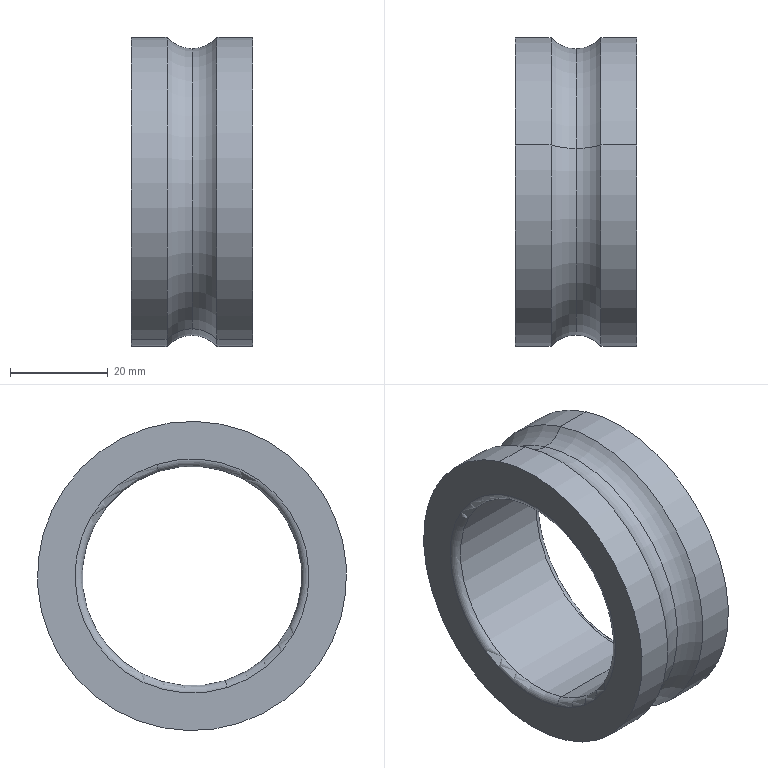Component | SolidWorks | UpperHousingAssembly-1_WormAxisAssembly-1_DeepGrooveBallBearing6309-1_BearingInnerRing-1 | 1 solid | 16 faces | box 25 x 63.4 x 63.4 mm | volume 35870 mm3 | torus 8 | cylinder 6 | plane 2 | commonest cylinder face diameters 63.4 x4 45 x2
build123d program:
from build123d import *

# Parameters (mm, degrees)
FILLET1_R = 1.5


with BuildPart() as part:
    # Sketch1 → Revolve1 (revolve)
    with BuildSketch(Plane.XY, mode=Mode.PRIVATE) as revolve1_sk:
        with BuildLine():
            Line((5.121, 31.7), (12.5, 31.7))
            Line((12.5, 31.7), (12.5, 22.5))
            Line((12.5, 22.5), (-12.5, 22.5))
            Line((-12.5, 22.5), (-12.5, 31.7))
            Line((-12.5, 31.7), (-5.121, 31.7))
            ThreePointArc((-5.121, 31.7), (0, 29.4), (5.121, 31.7))
        make_face()
    revolve(revolve1_sk.sketch.rotate(Axis((-18.919, 0, 0), (1, 0, 0)), 90), axis=Axis((-18.919, 0, 0), (1, 0, 0)))

    # Fillet1
    fillet1_edges = [part.edges().sort_by_distance(p)[0] for p in [
        (12.5, 0, -22.5),
        (-12.5, 0, -22.5),
    ]]
    fillet(fillet1_edges, radius=FILLET1_R)


solid = part.part

# Placed as in the assembly
solid = solid.moved(Location((1019.077, 1408.591, 1694.217), (0, 0, 0)))
STEP:
#1=COLOUR_RGB('',0.7922,0.8196,0.9333);
#2=FILL_AREA_STYLE_COLOUR('',#1);
#3=FILL_AREA_STYLE('',(#2));
#4=SURFACE_STYLE_FILL_AREA(#3);
#5=SURFACE_SIDE_STYLE('',(#4));
#6=SURFACE_STYLE_USAGE(.BOTH.,#5);
#7=PRESENTATION_STYLE_ASSIGNMENT((#6));
#8=CARTESIAN_POINT('',(39.92,55.834,67.891));
#9=VERTEX_POINT('',#8);
#10=CARTESIAN_POINT('',(40.121,55.806,67.805));
#11=VERTEX_POINT('',#10);
#12=CARTESIAN_POINT('',(40.121,55.888,68.062));
#13=DIRECTION('',(0.,-0.9532,0.3024));
#14=DIRECTION('',(0.,-0.3024,-0.9532));
#15=AXIS2_PLACEMENT_3D('',#12,#13,#14);
#16=CIRCLE('',#15,0.2697);
#17=EDGE_CURVE('',#9,#11,#16,.T.);
#18=ORIENTED_EDGE('',*,*,#17,.T.);
#19=CARTESIAN_POINT('',(40.121,55.106,65.598));
#20=VERTEX_POINT('',#19);
#21=CARTESIAN_POINT('',(40.121,55.456,66.701));
#22=DIRECTION('',(-1.,0.,0.));
#23=DIRECTION('',(0.,0.,1.));
#24=AXIS2_PLACEMENT_3D('',#21,#22,#23);
#25=CIRCLE('',#24,1.157);
#26=EDGE_CURVE('',#11,#20,#25,.T.);
#27=ORIENTED_EDGE('',*,*,#26,.T.);
#28=CARTESIAN_POINT('',(39.92,55.079,65.512));
#29=VERTEX_POINT('',#28);
#30=CARTESIAN_POINT('',(40.121,55.025,65.341));
#31=DIRECTION('',(0.,0.9532,-0.3024));
#32=DIRECTION('',(0.,0.3024,0.9532));
#33=AXIS2_PLACEMENT_3D('',#30,#31,#32);
#34=CIRCLE('',#33,0.2697);
#35=EDGE_CURVE('',#29,#20,#34,.T.);
#36=ORIENTED_EDGE('',*,*,#35,.F.);
#37=CARTESIAN_POINT('',(39.92,55.456,66.701));
#38=DIRECTION('',(-1.,0.,0.));
#39=DIRECTION('',(0.,0.3024,0.9532));
#40=AXIS2_PLACEMENT_3D('',#37,#38,#39);
#41=CIRCLE('',#40,1.248);
#42=EDGE_CURVE('',#9,#29,#41,.T.);
#43=ORIENTED_EDGE('',*,*,#42,.F.);
#44=EDGE_LOOP('',(#18,#27,#36,#43));
#45=FACE_OUTER_BOUND('',#44,.T.);
#46=CARTESIAN_POINT('',(40.121,55.456,66.701));
#47=DIRECTION('',(-1.,0.,0.));
#48=DIRECTION('',(0.,0.3024,0.9532));
#49=AXIS2_PLACEMENT_3D('',#46,#47,#48);
#50=TOROIDAL_SURFACE('',#49,1.427,0.2697);
#51=ADVANCED_FACE('',(#45),#50,.F.);
#52=ORIENTED_EDGE('',*,*,#35,.T.);
#53=CARTESIAN_POINT('',(40.121,55.456,66.701));
#54=DIRECTION('',(-1.,0.,0.));
#55=DIRECTION('',(0.,0.,1.));
#56=AXIS2_PLACEMENT_3D('',#53,#54,#55);
#57=CIRCLE('',#56,1.157);
#58=EDGE_CURVE('',#20,#11,#57,.T.);
#59=ORIENTED_EDGE('',*,*,#58,.T.);
#60=ORIENTED_EDGE('',*,*,#17,.F.);
#61=CARTESIAN_POINT('',(39.92,55.456,66.701));
#62=DIRECTION('',(-1.,0.,0.));
#63=DIRECTION('',(0.,0.3024,0.9532));
#64=AXIS2_PLACEMENT_3D('',#61,#62,#63);
#65=CIRCLE('',#64,1.248);
#66=EDGE_CURVE('',#29,#9,#65,.T.);
#67=ORIENTED_EDGE('',*,*,#66,.F.);
#68=EDGE_LOOP('',(#52,#59,#60,#67));
#69=FACE_OUTER_BOUND('',#68,.T.);
#70=CARTESIAN_POINT('',(40.121,55.456,66.701));
#71=DIRECTION('',(-1.,0.,0.));
#72=DIRECTION('',(0.,0.3024,0.9532));
#73=AXIS2_PLACEMENT_3D('',#70,#71,#72);
#74=TOROIDAL_SURFACE('',#73,1.427,0.2697);
#75=ADVANCED_FACE('',(#69),#74,.F.);
#76=CARTESIAN_POINT('',(40.554,55.188,65.857));
#77=VERTEX_POINT('',#76);
#78=CARTESIAN_POINT('',(40.554,55.724,67.546));
#79=VERTEX_POINT('',#78);
#80=CARTESIAN_POINT('',(40.554,55.456,66.701));
#81=DIRECTION('',(1.,0.,0.));
#82=DIRECTION('',(0.,0.3024,0.9532));
#83=AXIS2_PLACEMENT_3D('',#80,#81,#82);
#84=CIRCLE('',#83,0.8858);
#85=EDGE_CURVE('',#77,#79,#84,.T.);
#86=ORIENTED_EDGE('',*,*,#85,.F.);
#87=CARTESIAN_POINT('',(40.613,55.171,65.801));
#88=VERTEX_POINT('',#87);
#89=CARTESIAN_POINT('',(40.554,55.171,65.801));
#90=DIRECTION('',(0.,0.9532,-0.3024));
#91=DIRECTION('',(0.,0.3024,0.9532));
#92=AXIS2_PLACEMENT_3D('',#89,#90,#91);
#93=CIRCLE('',#92,0.05906);
#94=EDGE_CURVE('',#77,#88,#93,.T.);
#95=ORIENTED_EDGE('',*,*,#94,.T.);
#96=CARTESIAN_POINT('',(40.613,55.742,67.602));
#97=VERTEX_POINT('',#96);
#98=CARTESIAN_POINT('',(40.613,55.456,66.701));
#99=DIRECTION('',(-1.,0.,0.));
#100=DIRECTION('',(0.,0.3024,0.9532));
#101=AXIS2_PLACEMENT_3D('',#98,#99,#100);
#102=CIRCLE('',#101,0.9449);
#103=EDGE_CURVE('',#97,#88,#102,.T.);
#104=ORIENTED_EDGE('',*,*,#103,.F.);
#105=CARTESIAN_POINT('',(40.554,55.742,67.602));
#106=DIRECTION('',(0.,-0.9532,0.3024));
#107=DIRECTION('',(0.,-0.3024,-0.9532));
#108=AXIS2_PLACEMENT_3D('',#105,#106,#107);
#109=CIRCLE('',#108,0.05906);
#110=EDGE_CURVE('',#79,#97,#109,.T.);
#111=ORIENTED_EDGE('',*,*,#110,.F.);
#112=EDGE_LOOP('',(#86,#95,#104,#111));
#113=FACE_OUTER_BOUND('',#112,.T.);
#114=CARTESIAN_POINT('',(40.554,55.456,66.701));
#115=DIRECTION('',(-1.,0.,0.));
#116=DIRECTION('',(0.,0.3024,0.9532));
#117=AXIS2_PLACEMENT_3D('',#114,#115,#116);
#118=TOROIDAL_SURFACE('',#117,0.9449,0.05906);
#119=ADVANCED_FACE('',(#113),#118,.T.);
#120=CARTESIAN_POINT('',(39.688,55.724,67.546));
#121=VERTEX_POINT('',#120);
#122=CARTESIAN_POINT('',(39.688,55.188,65.857));
#123=VERTEX_POINT('',#122);
#124=CARTESIAN_POINT('',(39.688,55.456,66.701));
#125=DIRECTION('',(-1.,0.,0.));
#126=DIRECTION('',(0.,-0.3024,-0.9532));
#127=AXIS2_PLACEMENT_3D('',#124,#125,#126);
#128=CIRCLE('',#127,0.8858);
#129=EDGE_CURVE('',#121,#123,#128,.T.);
#130=ORIENTED_EDGE('',*,*,#129,.F.);
#131=CARTESIAN_POINT('',(39.629,55.742,67.602));
#132=VERTEX_POINT('',#131);
#133=CARTESIAN_POINT('',(39.688,55.742,67.602));
#134=DIRECTION('',(0.,0.9532,-0.3024));
#135=DIRECTION('',(0.,0.3024,0.9532));
#136=AXIS2_PLACEMENT_3D('',#133,#134,#135);
#137=CIRCLE('',#136,0.05906);
#138=EDGE_CURVE('',#121,#132,#137,.T.);
#139=ORIENTED_EDGE('',*,*,#138,.T.);
#140=CARTESIAN_POINT('',(39.629,55.171,65.801));
#141=VERTEX_POINT('',#140);
#142=CARTESIAN_POINT('',(39.629,55.456,66.701));
#143=DIRECTION('',(1.,0.,0.));
#144=DIRECTION('',(0.,-0.3024,-0.9532));
#145=AXIS2_PLACEMENT_3D('',#142,#143,#144);
#146=CIRCLE('',#145,0.9449);
#147=EDGE_CURVE('',#141,#132,#146,.T.);
#148=ORIENTED_EDGE('',*,*,#147,.F.);
#149=CARTESIAN_POINT('',(39.688,55.171,65.801));
#150=DIRECTION('',(0.,-0.9532,0.3024));
#151=DIRECTION('',(0.,-0.3024,-0.9532));
#152=AXIS2_PLACEMENT_3D('',#149,#150,#151);
#153=CIRCLE('',#152,0.05906);
#154=EDGE_CURVE('',#123,#141,#153,.T.);
#155=ORIENTED_EDGE('',*,*,#154,.F.);
#156=EDGE_LOOP('',(#130,#139,#148,#155));
#157=FACE_OUTER_BOUND('',#156,.T.);
#158=CARTESIAN_POINT('',(39.688,55.456,66.701));
#159=DIRECTION('',(1.,0.,0.));
#160=DIRECTION('',(0.,-0.3024,-0.9532));
#161=AXIS2_PLACEMENT_3D('',#158,#159,#160);
#162=TOROIDAL_SURFACE('',#161,0.9449,0.05906);
#163=ADVANCED_FACE('',(#157),#162,.T.);
#164=CARTESIAN_POINT('',(40.554,55.456,66.701));
#165=DIRECTION('',(1.,0.,0.));
#166=DIRECTION('',(0.,0.3024,0.9532));
#167=AXIS2_PLACEMENT_3D('',#164,#165,#166);
#168=CIRCLE('',#167,0.8858);
#169=EDGE_CURVE('',#79,#77,#168,.T.);
#170=ORIENTED_EDGE('',*,*,#169,.T.);
#171=CARTESIAN_POINT('',(39.376,55.188,65.857));
#172=DIRECTION('',(-1.,0.,0.));
#173=VECTOR('',#172,39.37);
#174=LINE('',#171,#173);
#175=EDGE_CURVE('',#77,#123,#174,.T.);
#176=ORIENTED_EDGE('',*,*,#175,.T.);
#177=CARTESIAN_POINT('',(39.688,55.456,66.701));
#178=DIRECTION('',(-1.,0.,0.));
#179=DIRECTION('',(0.,-0.3024,-0.9532));
#180=AXIS2_PLACEMENT_3D('',#177,#178,#179);
#181=CIRCLE('',#180,0.8858);
#182=EDGE_CURVE('',#123,#121,#181,.T.);
#183=ORIENTED_EDGE('',*,*,#182,.T.);
#184=CARTESIAN_POINT('',(39.376,55.724,67.546));
#185=DIRECTION('',(-1.,0.,0.));
#186=VECTOR('',#185,39.37);
#187=LINE('',#184,#186);
#188=EDGE_CURVE('',#79,#121,#187,.T.);
#189=ORIENTED_EDGE('',*,*,#188,.F.);
#190=EDGE_LOOP('',(#170,#176,#183,#189));
#191=FACE_OUTER_BOUND('',#190,.T.);
#192=CARTESIAN_POINT('',(39.376,55.456,66.701));
#193=DIRECTION('',(-1.,0.,0.));
#194=DIRECTION('',(0.,0.3024,0.9532));
#195=AXIS2_PLACEMENT_3D('',#192,#193,#194);
#196=CYLINDRICAL_SURFACE('',#195,0.8858);
#197=ADVANCED_FACE('',(#191),#196,.F.);
#198=ORIENTED_EDGE('',*,*,#42,.T.);
#199=CARTESIAN_POINT('',(39.629,55.079,65.512));
#200=VERTEX_POINT('',#199);
#201=CARTESIAN_POINT('',(39.376,55.079,65.512));
#202=DIRECTION('',(-1.,0.,0.));
#203=VECTOR('',#202,39.37);
#204=LINE('',#201,#203);
#205=EDGE_CURVE('',#29,#200,#204,.T.);
#206=ORIENTED_EDGE('',*,*,#205,.T.);
#207=CARTESIAN_POINT('',(39.629,55.834,67.891));
#208=VERTEX_POINT('',#207);
#209=CARTESIAN_POINT('',(39.629,55.456,66.701));
#210=DIRECTION('',(-1.,0.,0.));
#211=DIRECTION('',(0.,0.3024,0.9532));
#212=AXIS2_PLACEMENT_3D('',#209,#210,#211);
#213=CIRCLE('',#212,1.248);
#214=EDGE_CURVE('',#208,#200,#213,.T.);
#215=ORIENTED_EDGE('',*,*,#214,.F.);
#216=CARTESIAN_POINT('',(39.376,55.834,67.891));
#217=DIRECTION('',(-1.,0.,0.));
#218=VECTOR('',#217,39.37);
#219=LINE('',#216,#218);
#220=EDGE_CURVE('',#9,#208,#219,.T.);
#221=ORIENTED_EDGE('',*,*,#220,.F.);
#222=EDGE_LOOP('',(#198,#206,#215,#221));
#223=FACE_OUTER_BOUND('',#222,.T.);
#224=CARTESIAN_POINT('',(39.376,55.456,66.701));
#225=DIRECTION('',(-1.,0.,0.));
#226=DIRECTION('',(0.,0.3024,0.9532));
#227=AXIS2_PLACEMENT_3D('',#224,#225,#226);
#228=CYLINDRICAL_SURFACE('',#227,1.248);
#229=ADVANCED_FACE('',(#223),#228,.T.);
#230=ORIENTED_EDGE('',*,*,#58,.F.);
#231=CARTESIAN_POINT('',(40.323,55.079,65.512));
#232=VERTEX_POINT('',#231);
#233=CARTESIAN_POINT('',(40.121,55.025,65.341));
#234=DIRECTION('',(0.,0.9532,-0.3024));
#235=DIRECTION('',(0.,0.3024,0.9532));
#236=AXIS2_PLACEMENT_3D('',#233,#234,#235);
#237=CIRCLE('',#236,0.2697);
#238=EDGE_CURVE('',#20,#232,#237,.T.);
#239=ORIENTED_EDGE('',*,*,#238,.T.);
#240=CARTESIAN_POINT('',(40.323,55.834,67.891));
#241=VERTEX_POINT('',#240);
#242=CARTESIAN_POINT('',(40.323,55.456,66.701));
#243=DIRECTION('',(-1.,0.,0.));
#244=DIRECTION('',(0.,0.3024,0.9532));
#245=AXIS2_PLACEMENT_3D('',#242,#243,#244);
#246=CIRCLE('',#245,1.248);
#247=EDGE_CURVE('',#232,#241,#246,.T.);
#248=ORIENTED_EDGE('',*,*,#247,.T.);
#249=CARTESIAN_POINT('',(40.121,55.888,68.062));
#250=DIRECTION('',(0.,-0.9532,0.3024));
#251=DIRECTION('',(0.,-0.3024,-0.9532));
#252=AXIS2_PLACEMENT_3D('',#249,#250,#251);
#253=CIRCLE('',#252,0.2697);
#254=EDGE_CURVE('',#11,#241,#253,.T.);
#255=ORIENTED_EDGE('',*,*,#254,.F.);
#256=EDGE_LOOP('',(#230,#239,#248,#255));
#257=FACE_OUTER_BOUND('',#256,.T.);
#258=CARTESIAN_POINT('',(40.121,55.456,66.701));
#259=DIRECTION('',(-1.,0.,0.));
#260=DIRECTION('',(0.,0.3024,0.9532));
#261=AXIS2_PLACEMENT_3D('',#258,#259,#260);
#262=TOROIDAL_SURFACE('',#261,1.427,0.2697);
#263=ADVANCED_FACE('',(#257),#262,.F.);
#264=CARTESIAN_POINT('',(40.613,55.834,67.891));
#265=VERTEX_POINT('',#264);
#266=CARTESIAN_POINT('',(40.613,55.079,65.512));
#267=VERTEX_POINT('',#266);
#268=CARTESIAN_POINT('',(40.613,55.456,66.701));
#269=DIRECTION('',(-1.,0.,0.));
#270=DIRECTION('',(0.,0.3024,0.9532));
#271=AXIS2_PLACEMENT_3D('',#268,#269,#270);
#272=CIRCLE('',#271,1.248);
#273=EDGE_CURVE('',#265,#267,#272,.T.);
#274=ORIENTED_EDGE('',*,*,#273,.T.);
#275=CARTESIAN_POINT('',(39.376,55.079,65.512));
#276=DIRECTION('',(-1.,0.,0.));
#277=VECTOR('',#276,39.37);
#278=LINE('',#275,#277);
#279=EDGE_CURVE('',#267,#232,#278,.T.);
#280=ORIENTED_EDGE('',*,*,#279,.T.);
#281=CARTESIAN_POINT('',(40.323,55.456,66.701));
#282=DIRECTION('',(-1.,0.,0.));
#283=DIRECTION('',(0.,0.3024,0.9532));
#284=AXIS2_PLACEMENT_3D('',#281,#282,#283);
#285=CIRCLE('',#284,1.248);
#286=EDGE_CURVE('',#241,#232,#285,.T.);
#287=ORIENTED_EDGE('',*,*,#286,.F.);
#288=CARTESIAN_POINT('',(39.376,55.834,67.891));
#289=DIRECTION('',(-1.,0.,0.));
#290=VECTOR('',#289,39.37);
#291=LINE('',#288,#290);
#292=EDGE_CURVE('',#265,#241,#291,.T.);
#293=ORIENTED_EDGE('',*,*,#292,.F.);
#294=EDGE_LOOP('',(#274,#280,#287,#293));
#295=FACE_OUTER_BOUND('',#294,.T.);
#296=CARTESIAN_POINT('',(39.376,55.456,66.701));
#297=DIRECTION('',(-1.,0.,0.));
#298=DIRECTION('',(0.,0.3024,0.9532));
#299=AXIS2_PLACEMENT_3D('',#296,#297,#298);
#300=CYLINDRICAL_SURFACE('',#299,1.248);
#301=ADVANCED_FACE('',(#295),#300,.T.);
#302=ORIENTED_EDGE('',*,*,#103,.T.);
#303=CARTESIAN_POINT('',(40.613,55.456,66.701));
#304=DIRECTION('',(-1.,0.,0.));
#305=DIRECTION('',(0.,0.3024,0.9532));
#306=AXIS2_PLACEMENT_3D('',#303,#304,#305);
#307=CIRCLE('',#306,0.9449);
#308=EDGE_CURVE('',#88,#97,#307,.T.);
#309=ORIENTED_EDGE('',*,*,#308,.T.);
#310=EDGE_LOOP('',(#302,#309));
#311=FACE_BOUND('',#310,.T.);
#312=ORIENTED_EDGE('',*,*,#273,.F.);
#313=CARTESIAN_POINT('',(40.613,55.456,66.701));
#314=DIRECTION('',(-1.,0.,0.));
#315=DIRECTION('',(0.,0.3024,0.9532));
#316=AXIS2_PLACEMENT_3D('',#313,#314,#315);
#317=CIRCLE('',#316,1.248);
#318=EDGE_CURVE('',#267,#265,#317,.T.);
#319=ORIENTED_EDGE('',*,*,#318,.F.);
#320=EDGE_LOOP('',(#312,#319));
#321=FACE_OUTER_BOUND('',#320,.T.);
#322=CARTESIAN_POINT('',(40.613,56.301,66.434));
#323=DIRECTION('',(-1.,0.,0.));
#324=DIRECTION('',(0.,0.3024,0.9532));
#325=AXIS2_PLACEMENT_3D('',#322,#323,#324);
#326=PLANE('',#325);
#327=ADVANCED_FACE('',(#311,#321),#326,.F.);
#328=ORIENTED_EDGE('',*,*,#279,.F.);
#329=ORIENTED_EDGE('',*,*,#318,.T.);
#330=ORIENTED_EDGE('',*,*,#292,.T.);
#331=ORIENTED_EDGE('',*,*,#247,.F.);
#332=EDGE_LOOP('',(#328,#329,#330,#331));
#333=FACE_OUTER_BOUND('',#332,.T.);
#334=CARTESIAN_POINT('',(39.376,55.456,66.701));
#335=DIRECTION('',(-1.,0.,0.));
#336=DIRECTION('',(0.,0.3024,0.9532));
#337=AXIS2_PLACEMENT_3D('',#334,#335,#336);
#338=CYLINDRICAL_SURFACE('',#337,1.248);
#339=ADVANCED_FACE('',(#333),#338,.T.);
#340=ORIENTED_EDGE('',*,*,#26,.F.);
#341=ORIENTED_EDGE('',*,*,#254,.T.);
#342=ORIENTED_EDGE('',*,*,#286,.T.);
#343=ORIENTED_EDGE('',*,*,#238,.F.);
#344=EDGE_LOOP('',(#340,#341,#342,#343));
#345=FACE_OUTER_BOUND('',#344,.T.);
#346=CARTESIAN_POINT('',(40.121,55.456,66.701));
#347=DIRECTION('',(-1.,0.,0.));
#348=DIRECTION('',(0.,0.3024,0.9532));
#349=AXIS2_PLACEMENT_3D('',#346,#347,#348);
#350=TOROIDAL_SURFACE('',#349,1.427,0.2697);
#351=ADVANCED_FACE('',(#345),#350,.F.);
#352=ORIENTED_EDGE('',*,*,#205,.F.);
#353=ORIENTED_EDGE('',*,*,#66,.T.);
#354=ORIENTED_EDGE('',*,*,#220,.T.);
#355=CARTESIAN_POINT('',(39.629,55.456,66.701));
#356=DIRECTION('',(-1.,0.,0.));
#357=DIRECTION('',(0.,0.3024,0.9532));
#358=AXIS2_PLACEMENT_3D('',#355,#356,#357);
#359=CIRCLE('',#358,1.248);
#360=EDGE_CURVE('',#200,#208,#359,.T.);
#361=ORIENTED_EDGE('',*,*,#360,.F.);
#362=EDGE_LOOP('',(#352,#353,#354,#361));
#363=FACE_OUTER_BOUND('',#362,.T.);
#364=CARTESIAN_POINT('',(39.376,55.456,66.701));
#365=DIRECTION('',(-1.,0.,0.));
#366=DIRECTION('',(0.,0.3024,0.9532));
#367=AXIS2_PLACEMENT_3D('',#364,#365,#366);
#368=CYLINDRICAL_SURFACE('',#367,1.248);
#369=ADVANCED_FACE('',(#363),#368,.T.);
#370=ORIENTED_EDGE('',*,*,#147,.T.);
#371=CARTESIAN_POINT('',(39.629,55.456,66.701));
#372=DIRECTION('',(1.,0.,0.));
#373=DIRECTION('',(0.,-0.3024,-0.9532));
#374=AXIS2_PLACEMENT_3D('',#371,#372,#373);
#375=CIRCLE('',#374,0.9449);
#376=EDGE_CURVE('',#132,#141,#375,.T.);
#377=ORIENTED_EDGE('',*,*,#376,.T.);
#378=EDGE_LOOP('',(#370,#377));
#379=FACE_BOUND('',#378,.T.);
#380=ORIENTED_EDGE('',*,*,#214,.T.);
#381=ORIENTED_EDGE('',*,*,#360,.T.);
#382=EDGE_LOOP('',(#380,#381));
#383=FACE_OUTER_BOUND('',#382,.T.);
#384=CARTESIAN_POINT('',(39.629,56.301,66.434));
#385=DIRECTION('',(1.,0.,0.));
#386=DIRECTION('',(0.,-0.3024,-0.9532));
#387=AXIS2_PLACEMENT_3D('',#384,#385,#386);
#388=PLANE('',#387);
#389=ADVANCED_FACE('',(#379,#383),#388,.F.);
#390=ORIENTED_EDGE('',*,*,#175,.F.);
#391=ORIENTED_EDGE('',*,*,#85,.T.);
#392=ORIENTED_EDGE('',*,*,#188,.T.);
#393=ORIENTED_EDGE('',*,*,#129,.T.);
#394=EDGE_LOOP('',(#390,#391,#392,#393));
#395=FACE_OUTER_BOUND('',#394,.T.);
#396=CARTESIAN_POINT('',(39.376,55.456,66.701));
#397=DIRECTION('',(-1.,0.,0.));
#398=DIRECTION('',(0.,0.3024,0.9532));
#399=AXIS2_PLACEMENT_3D('',#396,#397,#398);
#400=CYLINDRICAL_SURFACE('',#399,0.8858);
#401=ADVANCED_FACE('',(#395),#400,.F.);
#402=ORIENTED_EDGE('',*,*,#138,.F.);
#403=ORIENTED_EDGE('',*,*,#182,.F.);
#404=ORIENTED_EDGE('',*,*,#154,.T.);
#405=ORIENTED_EDGE('',*,*,#376,.F.);
#406=EDGE_LOOP('',(#402,#403,#404,#405));
#407=FACE_OUTER_BOUND('',#406,.T.);
#408=CARTESIAN_POINT('',(39.688,55.456,66.701));
#409=DIRECTION('',(1.,0.,0.));
#410=DIRECTION('',(0.,-0.3024,-0.9532));
#411=AXIS2_PLACEMENT_3D('',#408,#409,#410);
#412=TOROIDAL_SURFACE('',#411,0.9449,0.05906);
#413=ADVANCED_FACE('',(#407),#412,.T.);
#414=ORIENTED_EDGE('',*,*,#94,.F.);
#415=ORIENTED_EDGE('',*,*,#169,.F.);
#416=ORIENTED_EDGE('',*,*,#110,.T.);
#417=ORIENTED_EDGE('',*,*,#308,.F.);
#418=EDGE_LOOP('',(#414,#415,#416,#417));
#419=FACE_OUTER_BOUND('',#418,.T.);
#420=CARTESIAN_POINT('',(40.554,55.456,66.701));
#421=DIRECTION('',(-1.,0.,0.));
#422=DIRECTION('',(0.,0.3024,0.9532));
#423=AXIS2_PLACEMENT_3D('',#420,#421,#422);
#424=TOROIDAL_SURFACE('',#423,0.9449,0.05906);
#425=ADVANCED_FACE('',(#419),#424,.T.);
#426=CLOSED_SHELL('',(#51,#75,#119,#163,#197,#229,#263,#301,#327,#339,#351,#369,#389,#401,#413,#425));
#427=MANIFOLD_SOLID_BREP('',#426);
#428=STYLED_ITEM('',(#7),#427);
#429=(LENGTH_UNIT()NAMED_UNIT(*)SI_UNIT($,.METRE.));
#430=LENGTH_MEASURE_WITH_UNIT(LENGTH_MEASURE(0.0254),#429);
#431=DIMENSIONAL_EXPONENTS(1.,0.,0.,0.,0.,0.,0.);
#432=(CONVERSION_BASED_UNIT('',#430)LENGTH_UNIT()NAMED_UNIT(#431));
#433=UNCERTAINTY_MEASURE_WITH_UNIT(LENGTH_MEASURE(0.00001),#432,'','');
#434=(NAMED_UNIT(*)PLANE_ANGLE_UNIT()SI_UNIT($,.RADIAN.));
#435=(NAMED_UNIT(*)SI_UNIT($,.STERADIAN.)SOLID_ANGLE_UNIT());
#436=(GEOMETRIC_REPRESENTATION_CONTEXT(3)GLOBAL_UNCERTAINTY_ASSIGNED_CONTEXT((#433))GLOBAL_UNIT_ASSIGNED_CONTEXT((#432,#434,#435))REPRESENTATION_CONTEXT('',''));
#437=MECHANICAL_DESIGN_GEOMETRIC_PRESENTATION_REPRESENTATION('',(#428),#436);
#438=CARTESIAN_POINT('',(0.,0.,0.));
#439=DIRECTION('',(0.,0.,1.));
#440=DIRECTION('',(1.,0.,0.));
#441=AXIS2_PLACEMENT_3D('',#438,#439,#440);
#442=(LENGTH_UNIT()NAMED_UNIT(*)SI_UNIT($,.METRE.));
#443=LENGTH_MEASURE_WITH_UNIT(LENGTH_MEASURE(0.0254),#442);
#444=DIMENSIONAL_EXPONENTS(1.,0.,0.,0.,0.,0.,0.);
#445=(CONVERSION_BASED_UNIT('',#443)LENGTH_UNIT()NAMED_UNIT(#444));
#446=UNCERTAINTY_MEASURE_WITH_UNIT(LENGTH_MEASURE(0.00001),#445,'','');
#447=(NAMED_UNIT(*)PLANE_ANGLE_UNIT()SI_UNIT($,.RADIAN.));
#448=(NAMED_UNIT(*)SI_UNIT($,.STERADIAN.)SOLID_ANGLE_UNIT());
#449=(GEOMETRIC_REPRESENTATION_CONTEXT(3)GLOBAL_UNCERTAINTY_ASSIGNED_CONTEXT((#446))GLOBAL_UNIT_ASSIGNED_CONTEXT((#445,#447,#448))REPRESENTATION_CONTEXT('',''));
#450=ADVANCED_BREP_SHAPE_REPRESENTATION('',(#427,#441),#449);
#451=PRESENTATION_LAYER_ASSIGNMENT('','',(#428));